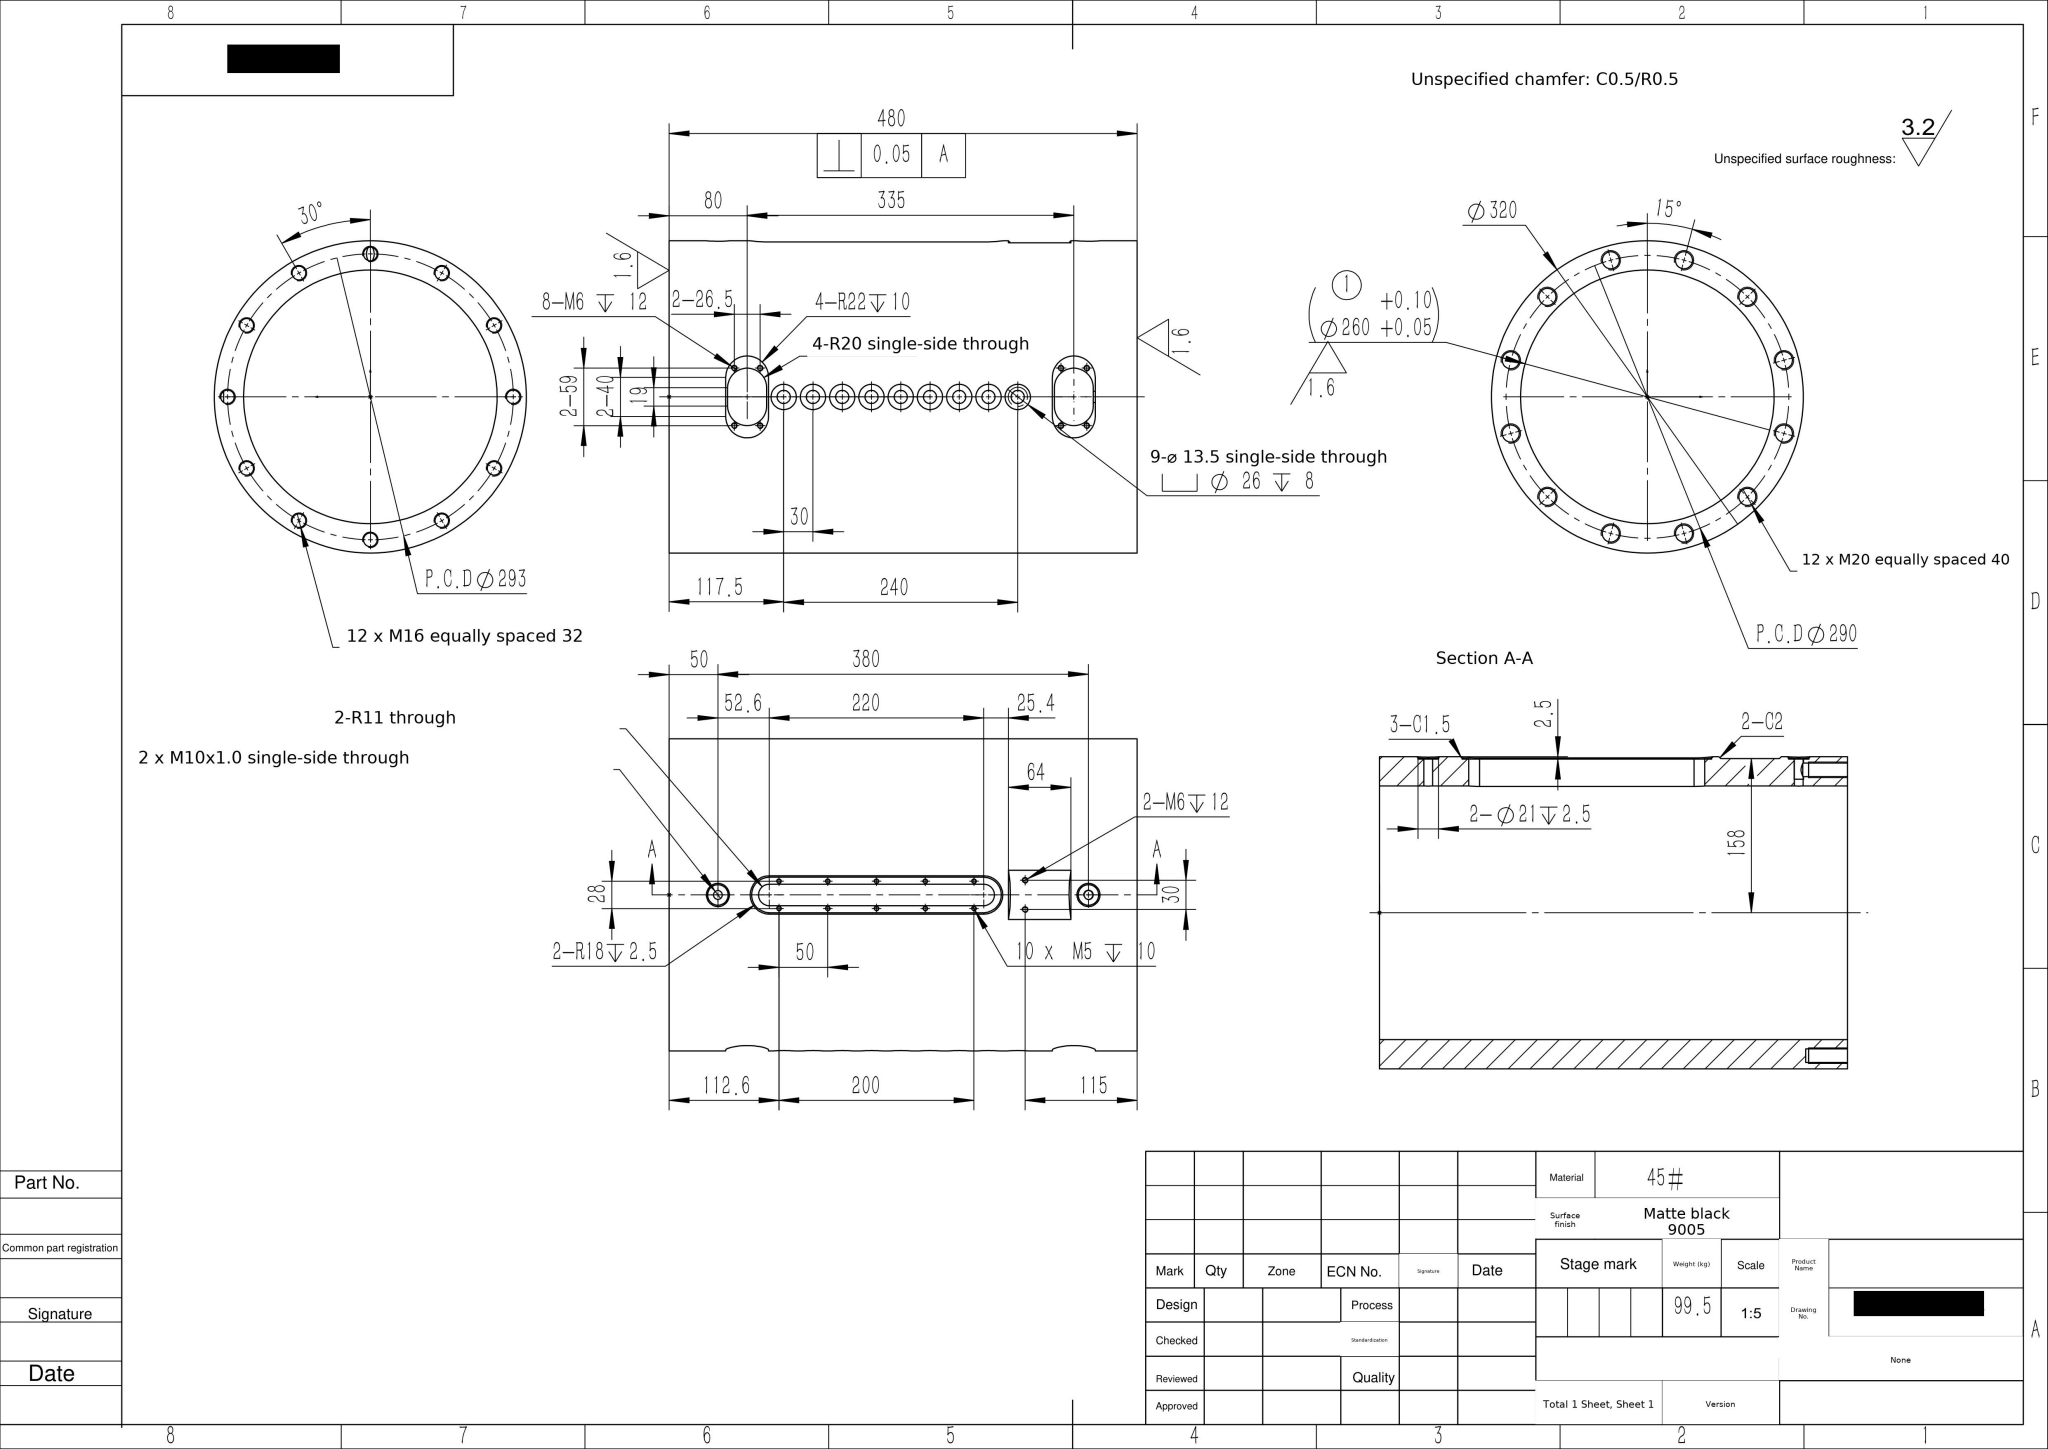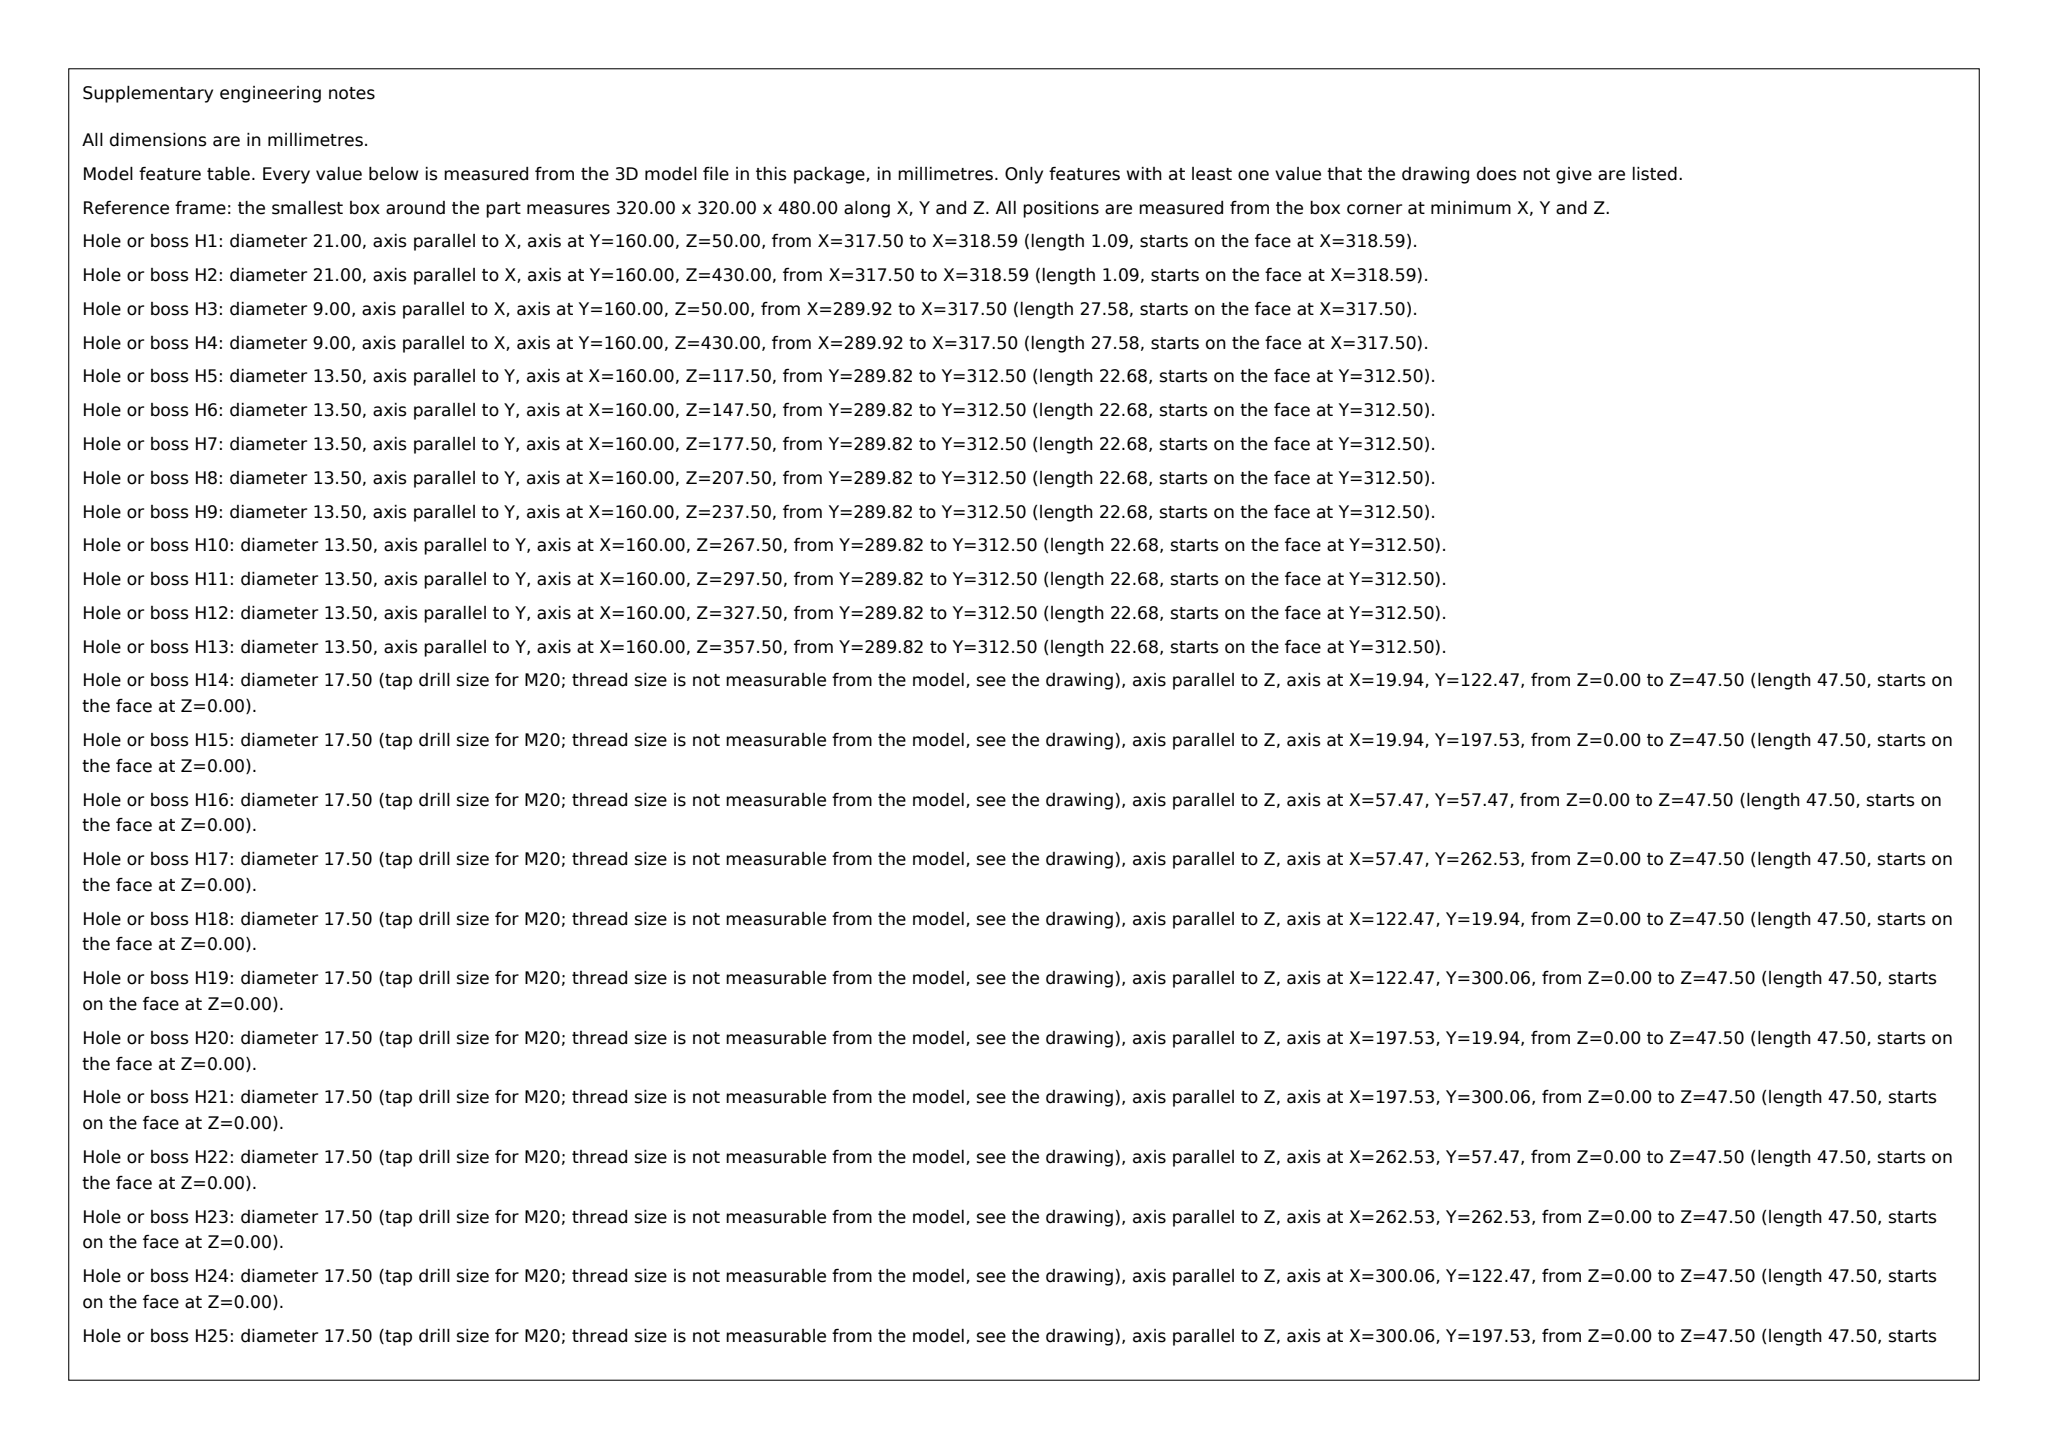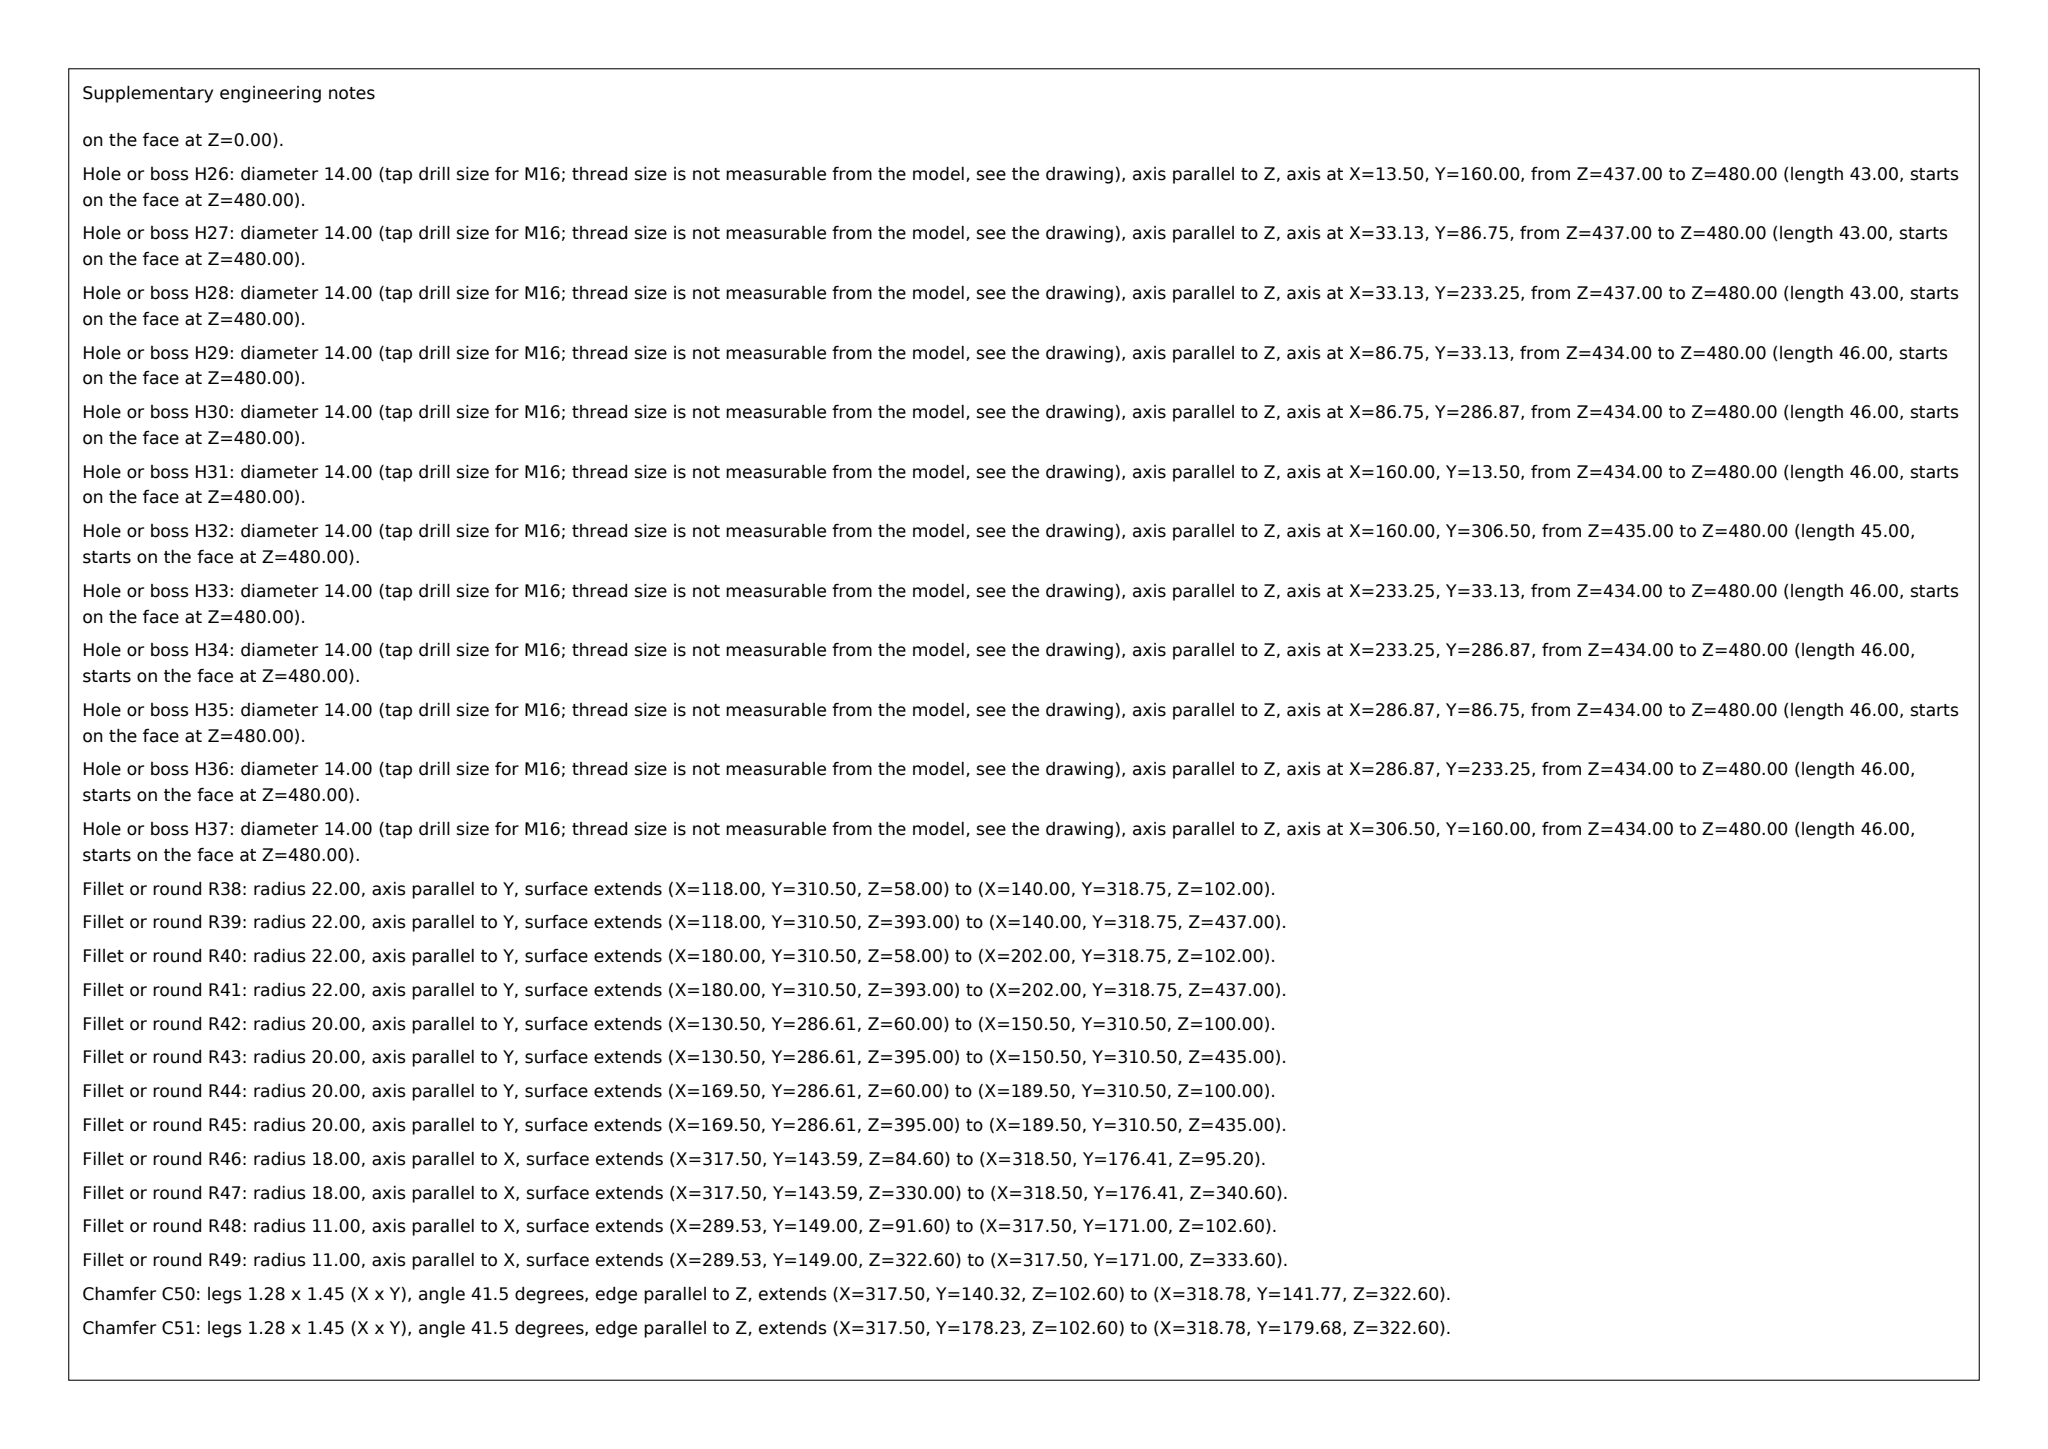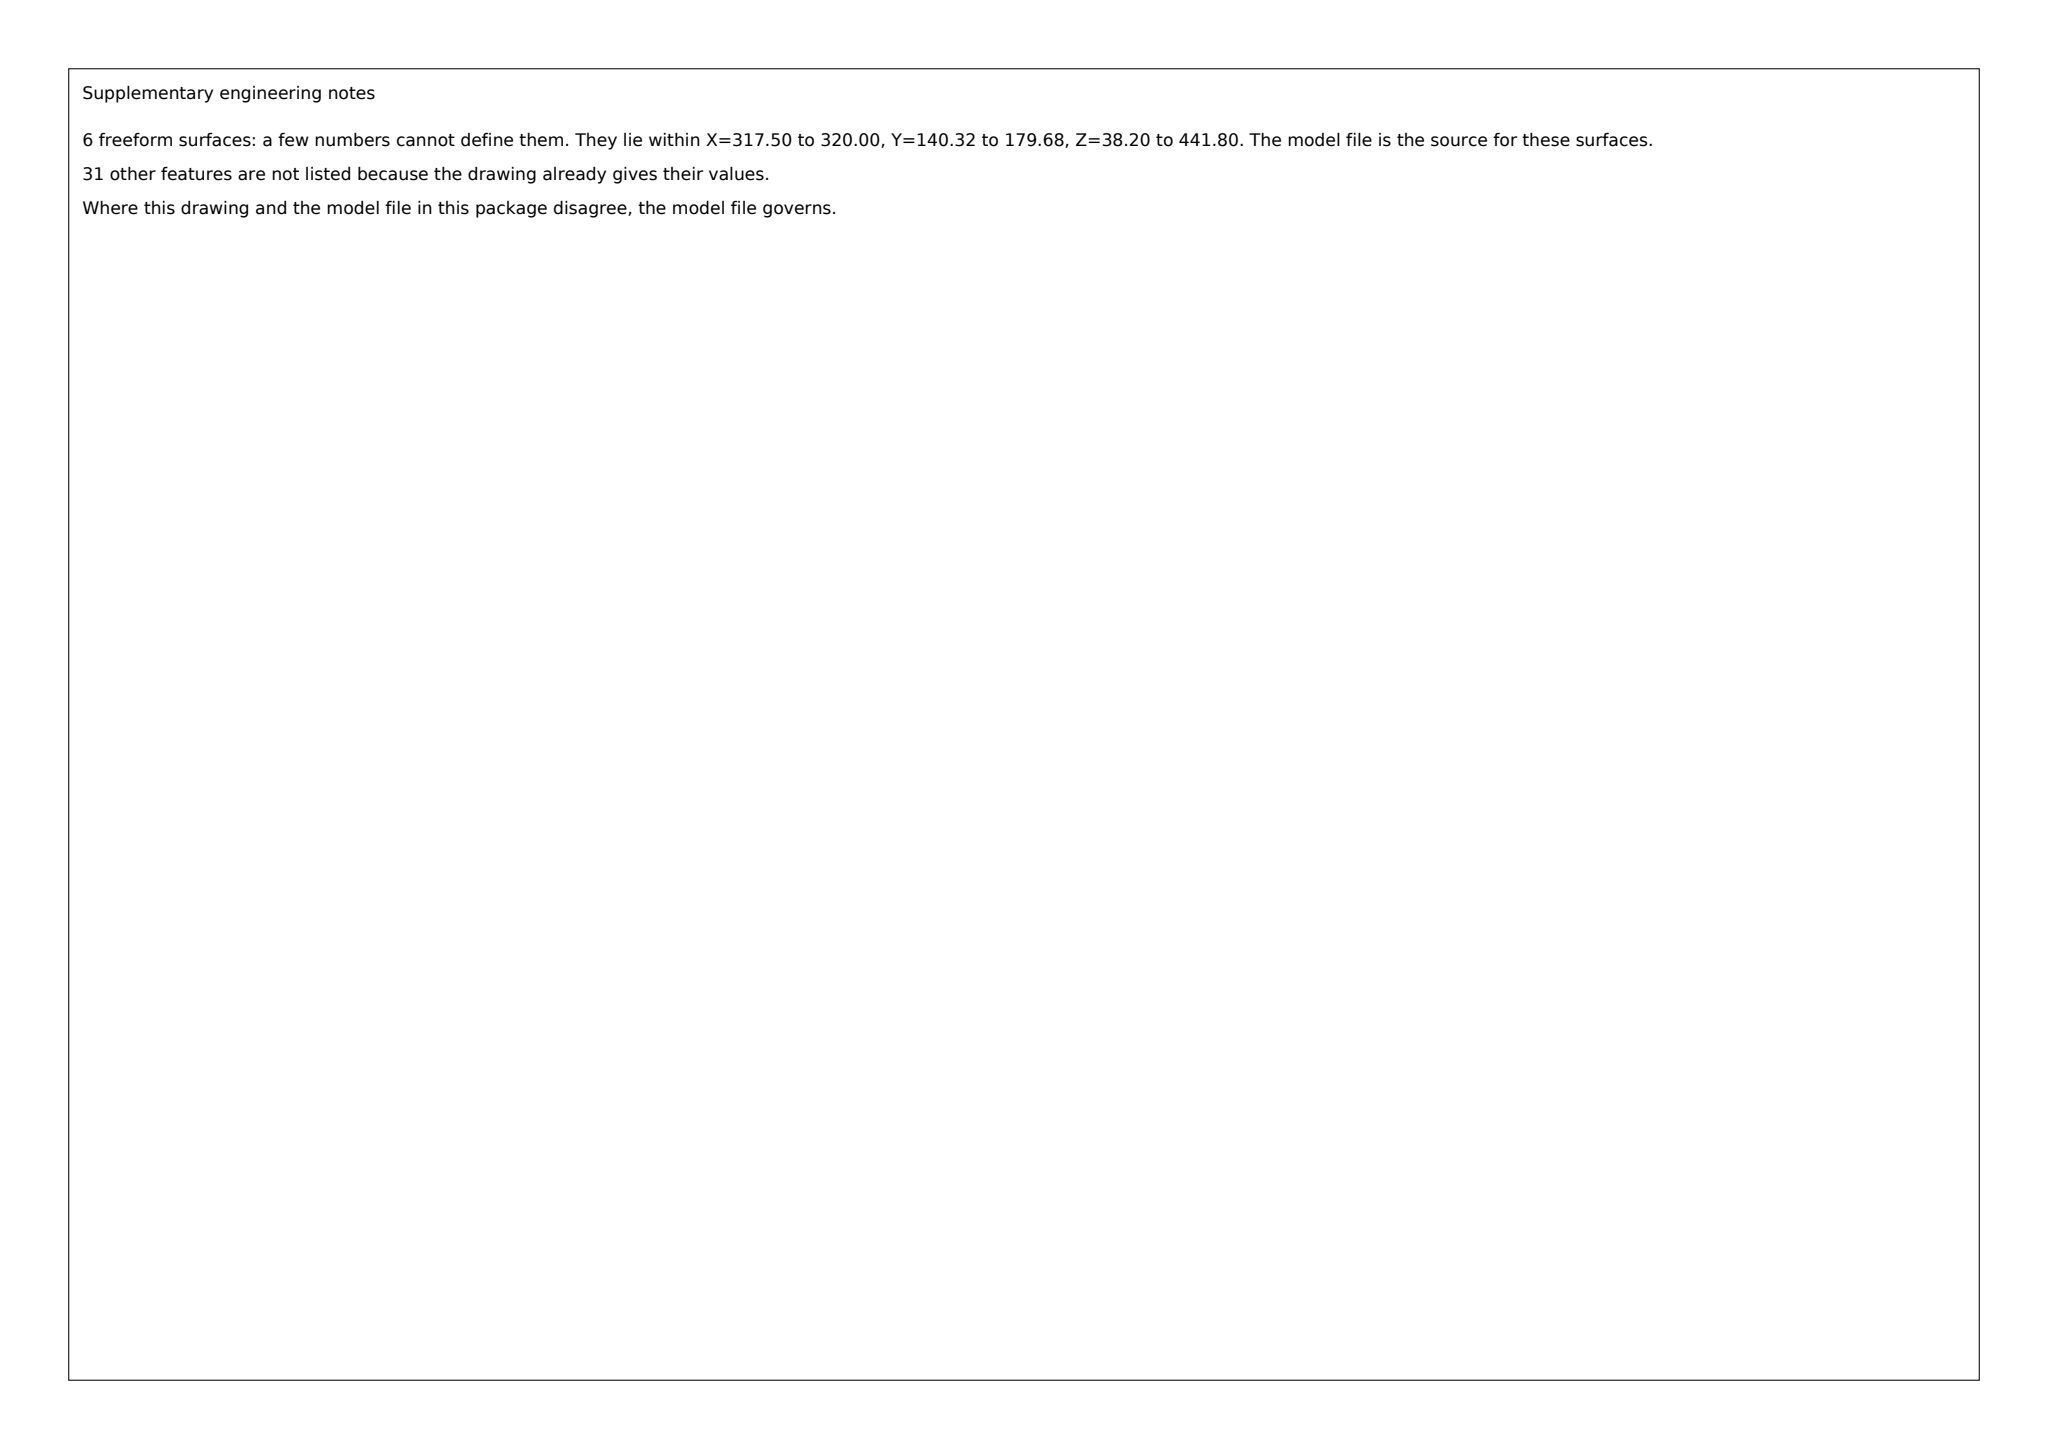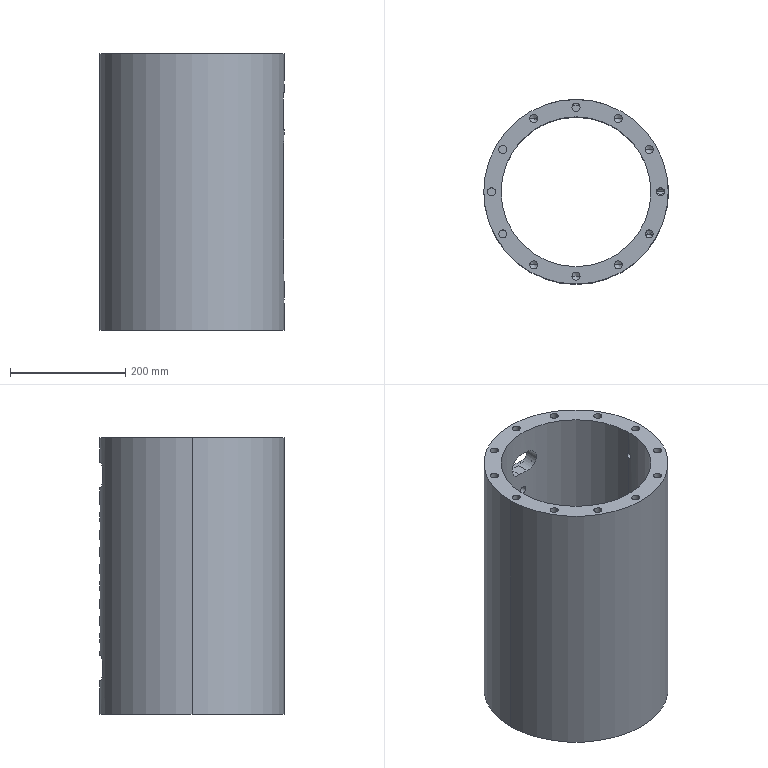Part | SolidWorks | mm | material 45# | 1 solid | 271 faces | box 320 x 320 x 480 mm | volume 12510495 mm3 | cylinder 150 | cone 83 | plane 32 | spline 6 | commonest cylinder face diameters 17.5 x24 14 x24 5 x20 4.2 x20 13.5 x18 26 x18 9 x4 21 x4